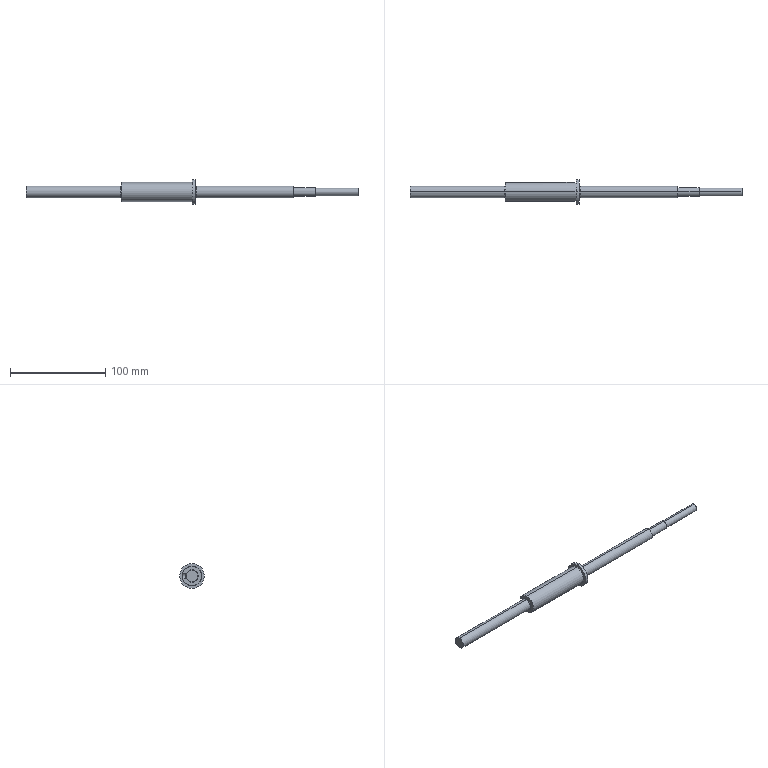Component | SolidWorks | LongAxis(Modified)-1 | 1 solid | 37 faces | box 349 x 26 x 26 mm | volume 50537 mm3 | cylinder 15 | plane 12 | torus 10 | commonest cylinder face diameters 12 x4 8 x2 26 x2 20 x2 9 x2 3 x2 6 x1 | material AISI 1045 Steel, Cold Drawn
STEP:
#1=CARTESIAN_POINT('',(-2.202,0.5951,13.465));
#2=VERTEX_POINT('',#1);
#3=CARTESIAN_POINT('',(-2.202,0.5951,14.016));
#4=VERTEX_POINT('',#3);
#5=CARTESIAN_POINT('',(-2.202,0.5951,13.74));
#6=DIRECTION('',(-1.,0.,0.));
#7=DIRECTION('',(0.,0.,1.));
#8=AXIS2_PLACEMENT_3D('',#5,#6,#7);
#9=CIRCLE('',#8,0.2756);
#10=EDGE_CURVE('',#2,#4,#9,.T.);
#11=ORIENTED_EDGE('',*,*,#10,.F.);
#12=CARTESIAN_POINT('',(-2.163,0.5951,13.504));
#13=VERTEX_POINT('',#12);
#14=CARTESIAN_POINT('',(-2.163,0.5951,13.465));
#15=DIRECTION('',(0.,1.,0.));
#16=DIRECTION('',(0.,0.,1.));
#17=AXIS2_PLACEMENT_3D('',#14,#15,#16);
#18=CIRCLE('',#17,0.03937);
#19=EDGE_CURVE('',#2,#13,#18,.T.);
#20=ORIENTED_EDGE('',*,*,#19,.T.);
#21=CARTESIAN_POINT('',(-2.163,0.5951,13.976));
#22=VERTEX_POINT('',#21);
#23=CARTESIAN_POINT('',(-2.163,0.5951,13.74));
#24=DIRECTION('',(1.,0.,0.));
#25=DIRECTION('',(0.,0.,1.));
#26=AXIS2_PLACEMENT_3D('',#23,#24,#25);
#27=CIRCLE('',#26,0.2362);
#28=EDGE_CURVE('',#22,#13,#27,.T.);
#29=ORIENTED_EDGE('',*,*,#28,.F.);
#30=CARTESIAN_POINT('',(-2.163,0.5951,14.016));
#31=DIRECTION('',(0.,-1.,0.));
#32=DIRECTION('',(0.,0.,-1.));
#33=AXIS2_PLACEMENT_3D('',#30,#31,#32);
#34=CIRCLE('',#33,0.03937);
#35=EDGE_CURVE('',#4,#22,#34,.T.);
#36=ORIENTED_EDGE('',*,*,#35,.F.);
#37=EDGE_LOOP('',(#11,#20,#29,#36));
#38=FACE_OUTER_BOUND('',#37,.T.);
#39=CARTESIAN_POINT('',(-2.163,0.5951,13.74));
#40=DIRECTION('',(-1.,0.,0.));
#41=DIRECTION('',(0.,0.,1.));
#42=AXIS2_PLACEMENT_3D('',#39,#40,#41);
#43=TOROIDAL_SURFACE('',#42,0.2756,0.03937);
#44=ADVANCED_FACE('',(#38),#43,.F.);
#45=CARTESIAN_POINT('',(1.853,0.5951,13.543));
#46=VERTEX_POINT('',#45);
#47=CARTESIAN_POINT('',(1.853,0.5951,13.937));
#48=VERTEX_POINT('',#47);
#49=CARTESIAN_POINT('',(1.853,0.5951,13.74));
#50=DIRECTION('',(-1.,0.,0.));
#51=DIRECTION('',(0.,0.,1.));
#52=AXIS2_PLACEMENT_3D('',#49,#50,#51);
#53=CIRCLE('',#52,0.1969);
#54=EDGE_CURVE('',#46,#48,#53,.T.);
#55=ORIENTED_EDGE('',*,*,#54,.F.);
#56=CARTESIAN_POINT('',(1.873,0.5951,13.563));
#57=VERTEX_POINT('',#56);
#58=CARTESIAN_POINT('',(1.873,0.5951,13.543));
#59=DIRECTION('',(0.,1.,0.));
#60=DIRECTION('',(0.,0.,1.));
#61=AXIS2_PLACEMENT_3D('',#58,#59,#60);
#62=CIRCLE('',#61,0.01969);
#63=EDGE_CURVE('',#46,#57,#62,.T.);
#64=ORIENTED_EDGE('',*,*,#63,.T.);
#65=CARTESIAN_POINT('',(1.873,0.5951,13.917));
#66=VERTEX_POINT('',#65);
#67=CARTESIAN_POINT('',(1.873,0.5951,13.74));
#68=DIRECTION('',(1.,0.,0.));
#69=DIRECTION('',(0.,0.,1.));
#70=AXIS2_PLACEMENT_3D('',#67,#68,#69);
#71=CIRCLE('',#70,0.1772);
#72=EDGE_CURVE('',#66,#57,#71,.T.);
#73=ORIENTED_EDGE('',*,*,#72,.F.);
#74=CARTESIAN_POINT('',(1.873,0.5951,13.937));
#75=DIRECTION('',(0.,-1.,0.));
#76=DIRECTION('',(0.,0.,-1.));
#77=AXIS2_PLACEMENT_3D('',#74,#75,#76);
#78=CIRCLE('',#77,0.01969);
#79=EDGE_CURVE('',#48,#66,#78,.T.);
#80=ORIENTED_EDGE('',*,*,#79,.F.);
#81=EDGE_LOOP('',(#55,#64,#73,#80));
#82=FACE_OUTER_BOUND('',#81,.T.);
#83=CARTESIAN_POINT('',(1.873,0.5951,13.74));
#84=DIRECTION('',(-1.,0.,0.));
#85=DIRECTION('',(0.,0.,1.));
#86=AXIS2_PLACEMENT_3D('',#83,#84,#85);
#87=TOROIDAL_SURFACE('',#86,0.1969,0.01969);
#88=ADVANCED_FACE('',(#82),#87,.F.);
#89=CARTESIAN_POINT('',(2.758,0.5951,13.563));
#90=VERTEX_POINT('',#89);
#91=CARTESIAN_POINT('',(2.758,0.5951,13.917));
#92=VERTEX_POINT('',#91);
#93=CARTESIAN_POINT('',(2.758,0.5951,13.74));
#94=DIRECTION('',(-1.,0.,0.));
#95=DIRECTION('',(0.,0.,1.));
#96=AXIS2_PLACEMENT_3D('',#93,#94,#95);
#97=CIRCLE('',#96,0.1772);
#98=EDGE_CURVE('',#90,#92,#97,.T.);
#99=ORIENTED_EDGE('',*,*,#98,.F.);
#100=CARTESIAN_POINT('',(2.778,0.5951,13.583));
#101=VERTEX_POINT('',#100);
#102=CARTESIAN_POINT('',(2.778,0.5951,13.563));
#103=DIRECTION('',(0.,1.,0.));
#104=DIRECTION('',(0.,0.,1.));
#105=AXIS2_PLACEMENT_3D('',#102,#103,#104);
#106=CIRCLE('',#105,0.01969);
#107=EDGE_CURVE('',#90,#101,#106,.T.);
#108=ORIENTED_EDGE('',*,*,#107,.T.);
#109=CARTESIAN_POINT('',(2.778,0.5951,13.898));
#110=VERTEX_POINT('',#109);
#111=CARTESIAN_POINT('',(2.778,0.5951,13.74));
#112=DIRECTION('',(1.,0.,0.));
#113=DIRECTION('',(0.,0.,1.));
#114=AXIS2_PLACEMENT_3D('',#111,#112,#113);
#115=CIRCLE('',#114,0.1575);
#116=EDGE_CURVE('',#110,#101,#115,.T.);
#117=ORIENTED_EDGE('',*,*,#116,.F.);
#118=CARTESIAN_POINT('',(2.778,0.5951,13.917));
#119=DIRECTION('',(0.,-1.,0.));
#120=DIRECTION('',(0.,0.,-1.));
#121=AXIS2_PLACEMENT_3D('',#118,#119,#120);
#122=CIRCLE('',#121,0.01969);
#123=EDGE_CURVE('',#92,#110,#122,.T.);
#124=ORIENTED_EDGE('',*,*,#123,.F.);
#125=EDGE_LOOP('',(#99,#108,#117,#124));
#126=FACE_OUTER_BOUND('',#125,.T.);
#127=CARTESIAN_POINT('',(2.778,0.5951,13.74));
#128=DIRECTION('',(-1.,0.,0.));
#129=DIRECTION('',(0.,0.,1.));
#130=AXIS2_PLACEMENT_3D('',#127,#128,#129);
#131=TOROIDAL_SURFACE('',#130,0.1772,0.01969);
#132=ADVANCED_FACE('',(#126),#131,.F.);
#133=CARTESIAN_POINT('',(-5.273,0.5951,13.996));
#134=VERTEX_POINT('',#133);
#135=CARTESIAN_POINT('',(-5.273,0.5951,13.484));
#136=VERTEX_POINT('',#135);
#137=CARTESIAN_POINT('',(-5.273,0.5951,13.74));
#138=DIRECTION('',(1.,0.,0.));
#139=DIRECTION('',(0.,0.,-1.));
#140=AXIS2_PLACEMENT_3D('',#137,#138,#139);
#141=CIRCLE('',#140,0.2559);
#142=EDGE_CURVE('',#134,#136,#141,.T.);
#143=ORIENTED_EDGE('',*,*,#142,.F.);
#144=CARTESIAN_POINT('',(-5.293,0.5951,13.976));
#145=VERTEX_POINT('',#144);
#146=CARTESIAN_POINT('',(-5.293,0.5951,13.996));
#147=DIRECTION('',(0.,1.,-0.));
#148=DIRECTION('',(0.,0.,1.));
#149=AXIS2_PLACEMENT_3D('',#146,#147,#148);
#150=CIRCLE('',#149,0.01969);
#151=EDGE_CURVE('',#134,#145,#150,.T.);
#152=ORIENTED_EDGE('',*,*,#151,.T.);
#153=CARTESIAN_POINT('',(-5.293,0.5951,13.504));
#154=VERTEX_POINT('',#153);
#155=CARTESIAN_POINT('',(-5.293,0.5951,13.74));
#156=DIRECTION('',(-1.,0.,0.));
#157=DIRECTION('',(0.,0.,-1.));
#158=AXIS2_PLACEMENT_3D('',#155,#156,#157);
#159=CIRCLE('',#158,0.2362);
#160=EDGE_CURVE('',#154,#145,#159,.T.);
#161=ORIENTED_EDGE('',*,*,#160,.F.);
#162=CARTESIAN_POINT('',(-5.293,0.5951,13.484));
#163=DIRECTION('',(0.,-1.,0.));
#164=DIRECTION('',(0.,0.,-1.));
#165=AXIS2_PLACEMENT_3D('',#162,#163,#164);
#166=CIRCLE('',#165,0.01969);
#167=EDGE_CURVE('',#136,#154,#166,.T.);
#168=ORIENTED_EDGE('',*,*,#167,.F.);
#169=EDGE_LOOP('',(#143,#152,#161,#168));
#170=FACE_OUTER_BOUND('',#169,.T.);
#171=CARTESIAN_POINT('',(-5.293,0.5951,13.74));
#172=DIRECTION('',(1.,0.,0.));
#173=DIRECTION('',(0.,0.,-1.));
#174=AXIS2_PLACEMENT_3D('',#171,#172,#173);
#175=TOROIDAL_SURFACE('',#174,0.2559,0.01969);
#176=ADVANCED_FACE('',(#170),#175,.F.);
#177=CARTESIAN_POINT('',(-2.32,0.5951,14.154));
#178=VERTEX_POINT('',#177);
#179=CARTESIAN_POINT('',(-2.32,0.5951,13.327));
#180=VERTEX_POINT('',#179);
#181=CARTESIAN_POINT('',(-2.32,0.5951,13.74));
#182=DIRECTION('',(1.,0.,0.));
#183=DIRECTION('',(0.,0.,-1.));
#184=AXIS2_PLACEMENT_3D('',#181,#182,#183);
#185=CIRCLE('',#184,0.4134);
#186=EDGE_CURVE('',#178,#180,#185,.T.);
#187=ORIENTED_EDGE('',*,*,#186,.F.);
#188=CARTESIAN_POINT('',(-2.34,0.5951,14.134));
#189=VERTEX_POINT('',#188);
#190=CARTESIAN_POINT('',(-2.34,0.5951,14.154));
#191=DIRECTION('',(0.,1.,-0.));
#192=DIRECTION('',(0.,0.,1.));
#193=AXIS2_PLACEMENT_3D('',#190,#191,#192);
#194=CIRCLE('',#193,0.01969);
#195=EDGE_CURVE('',#178,#189,#194,.T.);
#196=ORIENTED_EDGE('',*,*,#195,.T.);
#197=CARTESIAN_POINT('',(-2.34,0.5951,13.346));
#198=VERTEX_POINT('',#197);
#199=CARTESIAN_POINT('',(-2.34,0.5951,13.74));
#200=DIRECTION('',(-1.,0.,0.));
#201=DIRECTION('',(0.,0.,-1.));
#202=AXIS2_PLACEMENT_3D('',#199,#200,#201);
#203=CIRCLE('',#202,0.3937);
#204=EDGE_CURVE('',#198,#189,#203,.T.);
#205=ORIENTED_EDGE('',*,*,#204,.F.);
#206=CARTESIAN_POINT('',(-2.34,0.5951,13.327));
#207=DIRECTION('',(0.,-1.,0.));
#208=DIRECTION('',(0.,0.,-1.));
#209=AXIS2_PLACEMENT_3D('',#206,#207,#208);
#210=CIRCLE('',#209,0.01969);
#211=EDGE_CURVE('',#180,#198,#210,.T.);
#212=ORIENTED_EDGE('',*,*,#211,.F.);
#213=EDGE_LOOP('',(#187,#196,#205,#212));
#214=FACE_OUTER_BOUND('',#213,.T.);
#215=CARTESIAN_POINT('',(-2.34,0.5951,13.74));
#216=DIRECTION('',(1.,0.,0.));
#217=DIRECTION('',(0.,0.,-1.));
#218=AXIS2_PLACEMENT_3D('',#215,#216,#217);
#219=TOROIDAL_SURFACE('',#218,0.4134,0.01969);
#220=ADVANCED_FACE('',(#214),#219,.F.);
#221=CARTESIAN_POINT('',(4.53,0.5951,13.898));
#222=VERTEX_POINT('',#221);
#223=CARTESIAN_POINT('',(4.53,0.5951,13.583));
#224=VERTEX_POINT('',#223);
#225=CARTESIAN_POINT('',(4.53,0.5951,13.74));
#226=DIRECTION('',(-1.,0.,0.));
#227=DIRECTION('',(0.,0.,1.));
#228=AXIS2_PLACEMENT_3D('',#225,#226,#227);
#229=CIRCLE('',#228,0.1575);
#230=EDGE_CURVE('',#222,#224,#229,.T.);
#231=ORIENTED_EDGE('',*,*,#230,.T.);
#232=CARTESIAN_POINT('',(-9.21,0.5951,13.583));
#233=DIRECTION('',(-1.,0.,0.));
#234=VECTOR('',#233,39.37);
#235=LINE('',#232,#234);
#236=EDGE_CURVE('',#224,#101,#235,.T.);
#237=ORIENTED_EDGE('',*,*,#236,.T.);
#238=CARTESIAN_POINT('',(2.778,0.5951,13.74));
#239=DIRECTION('',(1.,0.,0.));
#240=DIRECTION('',(0.,0.,1.));
#241=AXIS2_PLACEMENT_3D('',#238,#239,#240);
#242=CIRCLE('',#241,0.1575);
#243=EDGE_CURVE('',#101,#110,#242,.T.);
#244=ORIENTED_EDGE('',*,*,#243,.T.);
#245=CARTESIAN_POINT('',(-9.21,0.5951,13.898));
#246=DIRECTION('',(-1.,0.,0.));
#247=VECTOR('',#246,39.37);
#248=LINE('',#245,#247);
#249=EDGE_CURVE('',#222,#110,#248,.T.);
#250=ORIENTED_EDGE('',*,*,#249,.F.);
#251=EDGE_LOOP('',(#231,#237,#244,#250));
#252=FACE_OUTER_BOUND('',#251,.T.);
#253=CARTESIAN_POINT('',(-9.21,0.5951,13.74));
#254=DIRECTION('',(-1.,0.,0.));
#255=DIRECTION('',(0.,0.,1.));
#256=AXIS2_PLACEMENT_3D('',#253,#254,#255);
#257=CYLINDRICAL_SURFACE('',#256,0.1575);
#258=ADVANCED_FACE('',(#252),#257,.T.);
#259=CARTESIAN_POINT('',(1.853,0.5951,13.976));
#260=VERTEX_POINT('',#259);
#261=CARTESIAN_POINT('',(1.853,0.5951,13.504));
#262=VERTEX_POINT('',#261);
#263=CARTESIAN_POINT('',(1.853,0.5951,13.74));
#264=DIRECTION('',(-1.,0.,0.));
#265=DIRECTION('',(0.,0.,1.));
#266=AXIS2_PLACEMENT_3D('',#263,#264,#265);
#267=CIRCLE('',#266,0.2362);
#268=EDGE_CURVE('',#260,#262,#267,.T.);
#269=ORIENTED_EDGE('',*,*,#268,.T.);
#270=CARTESIAN_POINT('',(-9.21,0.5951,13.504));
#271=DIRECTION('',(-1.,0.,0.));
#272=VECTOR('',#271,39.37);
#273=LINE('',#270,#272);
#274=EDGE_CURVE('',#262,#13,#273,.T.);
#275=ORIENTED_EDGE('',*,*,#274,.T.);
#276=CARTESIAN_POINT('',(-2.163,0.5951,13.74));
#277=DIRECTION('',(1.,0.,0.));
#278=DIRECTION('',(0.,0.,1.));
#279=AXIS2_PLACEMENT_3D('',#276,#277,#278);
#280=CIRCLE('',#279,0.2362);
#281=EDGE_CURVE('',#13,#22,#280,.T.);
#282=ORIENTED_EDGE('',*,*,#281,.T.);
#283=CARTESIAN_POINT('',(-9.21,0.5951,13.976));
#284=DIRECTION('',(-1.,0.,0.));
#285=VECTOR('',#284,39.37);
#286=LINE('',#283,#285);
#287=EDGE_CURVE('',#260,#22,#286,.T.);
#288=ORIENTED_EDGE('',*,*,#287,.F.);
#289=EDGE_LOOP('',(#269,#275,#282,#288));
#290=FACE_OUTER_BOUND('',#289,.T.);
#291=CARTESIAN_POINT('',(-9.21,0.5951,13.74));
#292=DIRECTION('',(-1.,0.,0.));
#293=DIRECTION('',(0.,0.,1.));
#294=AXIS2_PLACEMENT_3D('',#291,#292,#293);
#295=CYLINDRICAL_SURFACE('',#294,0.2362);
#296=ADVANCED_FACE('',(#290),#295,.T.);
#297=CARTESIAN_POINT('',(-2.202,0.5951,14.252));
#298=VERTEX_POINT('',#297);
#299=CARTESIAN_POINT('',(-2.202,0.5951,13.228));
#300=VERTEX_POINT('',#299);
#301=CARTESIAN_POINT('',(-2.202,0.5951,13.74));
#302=DIRECTION('',(-1.,0.,0.));
#303=DIRECTION('',(0.,0.,1.));
#304=AXIS2_PLACEMENT_3D('',#301,#302,#303);
#305=CIRCLE('',#304,0.5118);
#306=EDGE_CURVE('',#298,#300,#305,.T.);
#307=ORIENTED_EDGE('',*,*,#306,.T.);
#308=CARTESIAN_POINT('',(-2.32,0.5951,13.228));
#309=VERTEX_POINT('',#308);
#310=CARTESIAN_POINT('',(-9.21,0.5951,13.228));
#311=DIRECTION('',(-1.,0.,0.));
#312=VECTOR('',#311,39.37);
#313=LINE('',#310,#312);
#314=EDGE_CURVE('',#300,#309,#313,.T.);
#315=ORIENTED_EDGE('',*,*,#314,.T.);
#316=CARTESIAN_POINT('',(-2.32,0.5951,14.252));
#317=VERTEX_POINT('',#316);
#318=CARTESIAN_POINT('',(-2.32,0.5951,13.74));
#319=DIRECTION('',(-1.,0.,0.));
#320=DIRECTION('',(0.,0.,1.));
#321=AXIS2_PLACEMENT_3D('',#318,#319,#320);
#322=CIRCLE('',#321,0.5118);
#323=EDGE_CURVE('',#317,#309,#322,.T.);
#324=ORIENTED_EDGE('',*,*,#323,.F.);
#325=CARTESIAN_POINT('',(-9.21,0.5951,14.252));
#326=DIRECTION('',(-1.,0.,0.));
#327=VECTOR('',#326,39.37);
#328=LINE('',#325,#327);
#329=EDGE_CURVE('',#298,#317,#328,.T.);
#330=ORIENTED_EDGE('',*,*,#329,.F.);
#331=EDGE_LOOP('',(#307,#315,#324,#330));
#332=FACE_OUTER_BOUND('',#331,.T.);
#333=CARTESIAN_POINT('',(-9.21,0.5951,13.74));
#334=DIRECTION('',(-1.,0.,0.));
#335=DIRECTION('',(0.,0.,1.));
#336=AXIS2_PLACEMENT_3D('',#333,#334,#335);
#337=CYLINDRICAL_SURFACE('',#336,0.5118);
#338=ADVANCED_FACE('',(#332),#337,.T.);
#339=CARTESIAN_POINT('',(-5.293,0.5951,13.74));
#340=DIRECTION('',(-1.,0.,0.));
#341=DIRECTION('',(0.,0.,-1.));
#342=AXIS2_PLACEMENT_3D('',#339,#340,#341);
#343=CIRCLE('',#342,0.2362);
#344=EDGE_CURVE('',#145,#154,#343,.T.);
#345=ORIENTED_EDGE('',*,*,#344,.T.);
#346=CARTESIAN_POINT('',(-9.21,0.5951,13.504));
#347=VERTEX_POINT('',#346);
#348=CARTESIAN_POINT('',(-9.21,0.5951,13.504));
#349=DIRECTION('',(-1.,0.,0.));
#350=VECTOR('',#349,39.37);
#351=LINE('',#348,#350);
#352=EDGE_CURVE('',#154,#347,#351,.T.);
#353=ORIENTED_EDGE('',*,*,#352,.T.);
#354=CARTESIAN_POINT('',(-9.21,0.5951,13.976));
#355=VERTEX_POINT('',#354);
#356=CARTESIAN_POINT('',(-9.21,0.5951,13.74));
#357=DIRECTION('',(-1.,0.,0.));
#358=DIRECTION('',(0.,0.,1.));
#359=AXIS2_PLACEMENT_3D('',#356,#357,#358);
#360=CIRCLE('',#359,0.2362);
#361=EDGE_CURVE('',#355,#347,#360,.T.);
#362=ORIENTED_EDGE('',*,*,#361,.F.);
#363=CARTESIAN_POINT('',(-9.21,0.5951,13.976));
#364=DIRECTION('',(-1.,0.,0.));
#365=VECTOR('',#364,39.37);
#366=LINE('',#363,#365);
#367=EDGE_CURVE('',#145,#355,#366,.T.);
#368=ORIENTED_EDGE('',*,*,#367,.F.);
#369=EDGE_LOOP('',(#345,#353,#362,#368));
#370=FACE_OUTER_BOUND('',#369,.T.);
#371=CARTESIAN_POINT('',(-9.21,0.5951,13.74));
#372=DIRECTION('',(-1.,0.,0.));
#373=DIRECTION('',(0.,0.,1.));
#374=AXIS2_PLACEMENT_3D('',#371,#372,#373);
#375=CYLINDRICAL_SURFACE('',#374,0.2362);
#376=ADVANCED_FACE('',(#370),#375,.T.);
#377=CARTESIAN_POINT('',(-2.34,0.5951,13.74));
#378=DIRECTION('',(-1.,0.,0.));
#379=DIRECTION('',(0.,0.,-1.));
#380=AXIS2_PLACEMENT_3D('',#377,#378,#379);
#381=CIRCLE('',#380,0.3937);
#382=EDGE_CURVE('',#189,#198,#381,.T.);
#383=ORIENTED_EDGE('',*,*,#382,.T.);
#384=CARTESIAN_POINT('',(-5.273,0.5951,13.346));
#385=VERTEX_POINT('',#384);
#386=CARTESIAN_POINT('',(-9.21,0.5951,13.346));
#387=DIRECTION('',(-1.,0.,0.));
#388=VECTOR('',#387,39.37);
#389=LINE('',#386,#388);
#390=EDGE_CURVE('',#198,#385,#389,.T.);
#391=ORIENTED_EDGE('',*,*,#390,.T.);
#392=CARTESIAN_POINT('',(-5.273,0.9707,13.622));
#393=VERTEX_POINT('',#392);
#394=CARTESIAN_POINT('',(-5.273,0.5951,13.74));
#395=DIRECTION('',(-1.,0.,0.));
#396=DIRECTION('',(0.,0.,1.));
#397=AXIS2_PLACEMENT_3D('',#394,#395,#396);
#398=CIRCLE('',#397,0.3937);
#399=EDGE_CURVE('',#393,#385,#398,.T.);
#400=ORIENTED_EDGE('',*,*,#399,.F.);
#401=CARTESIAN_POINT('',(-2.911,0.9707,13.622));
#402=VERTEX_POINT('',#401);
#403=CARTESIAN_POINT('',(-9.21,0.9707,13.622));
#404=DIRECTION('',(-1.,0.,0.));
#405=VECTOR('',#404,39.37);
#406=LINE('',#403,#405);
#407=EDGE_CURVE('',#402,#393,#406,.T.);
#408=ORIENTED_EDGE('',*,*,#407,.F.);
#409=CARTESIAN_POINT('',(-2.911,0.9707,13.858));
#410=VERTEX_POINT('',#409);
#411=CARTESIAN_POINT('',(-2.911,0.9707,13.858));
#412=CARTESIAN_POINT('',(-2.903,0.9707,13.858));
#413=CARTESIAN_POINT('',(-2.895,0.9709,13.857));
#414=CARTESIAN_POINT('',(-2.88,0.9718,13.854));
#415=CARTESIAN_POINT('',(-2.873,0.9725,13.852));
#416=CARTESIAN_POINT('',(-2.858,0.9743,13.846));
#417=CARTESIAN_POINT('',(-2.852,0.9753,13.843));
#418=CARTESIAN_POINT('',(-2.839,0.9775,13.834));
#419=CARTESIAN_POINT('',(-2.833,0.9787,13.829));
#420=CARTESIAN_POINT('',(-2.817,0.9822,13.813));
#421=CARTESIAN_POINT('',(-2.808,0.9845,13.8));
#422=CARTESIAN_POINT('',(-2.799,0.987,13.778));
#423=CARTESIAN_POINT('',(-2.797,0.9877,13.771));
#424=CARTESIAN_POINT('',(-2.794,0.9886,13.756));
#425=CARTESIAN_POINT('',(-2.793,0.9888,13.748));
#426=CARTESIAN_POINT('',(-2.793,0.9888,13.733));
#427=CARTESIAN_POINT('',(-2.794,0.9886,13.725));
#428=CARTESIAN_POINT('',(-2.797,0.9877,13.709));
#429=CARTESIAN_POINT('',(-2.799,0.987,13.702));
#430=CARTESIAN_POINT('',(-2.805,0.9854,13.688));
#431=CARTESIAN_POINT('',(-2.808,0.9844,13.681));
#432=CARTESIAN_POINT('',(-2.817,0.9822,13.668));
#433=CARTESIAN_POINT('',(-2.822,0.981,13.662));
#434=CARTESIAN_POINT('',(-2.833,0.9787,13.651));
#435=CARTESIAN_POINT('',(-2.839,0.9775,13.646));
#436=CARTESIAN_POINT('',(-2.852,0.9753,13.638));
#437=CARTESIAN_POINT('',(-2.858,0.9743,13.634));
#438=CARTESIAN_POINT('',(-2.873,0.9726,13.628));
#439=CARTESIAN_POINT('',(-2.88,0.9719,13.626));
#440=CARTESIAN_POINT('',(-2.895,0.9709,13.623));
#441=CARTESIAN_POINT('',(-2.903,0.9707,13.622));
#442=CARTESIAN_POINT('',(-2.911,0.9707,13.622));
#443=B_SPLINE_CURVE_WITH_KNOTS('',3,(#411,#412,#413,#414,#415,#416,#417,#418,#419,#420,#421,#422,#423,#424,#425,#426,#427,#428,#429,#430,#431,#432,#433,#434,#435,#436,#437,#438,#439,#440,#441,#442),.UNSPECIFIED.,.F.,.F.,(4,2,2,2,2,2,2,2,2,2,2,2,2,2,2,4),(0.,0.0005894,0.001179,0.001768,0.002358,0.003536,0.004126,0.004715,0.005305,0.005894,0.006484,0.007073,0.007662,0.008252,0.008841,0.009431),.UNSPECIFIED.);
#444=EDGE_CURVE('',#410,#402,#443,.T.);
#445=ORIENTED_EDGE('',*,*,#444,.F.);
#446=CARTESIAN_POINT('',(-5.273,0.9707,13.858));
#447=VERTEX_POINT('',#446);
#448=CARTESIAN_POINT('',(-9.21,0.9707,13.858));
#449=DIRECTION('',(1.,0.,0.));
#450=VECTOR('',#449,39.37);
#451=LINE('',#448,#450);
#452=EDGE_CURVE('',#447,#410,#451,.T.);
#453=ORIENTED_EDGE('',*,*,#452,.F.);
#454=CARTESIAN_POINT('',(-5.273,0.5951,14.134));
#455=VERTEX_POINT('',#454);
#456=CARTESIAN_POINT('',(-5.273,0.5951,13.74));
#457=DIRECTION('',(-1.,0.,0.));
#458=DIRECTION('',(0.,0.,1.));
#459=AXIS2_PLACEMENT_3D('',#456,#457,#458);
#460=CIRCLE('',#459,0.3937);
#461=EDGE_CURVE('',#455,#447,#460,.T.);
#462=ORIENTED_EDGE('',*,*,#461,.F.);
#463=CARTESIAN_POINT('',(-9.21,0.5951,14.134));
#464=DIRECTION('',(-1.,0.,0.));
#465=VECTOR('',#464,39.37);
#466=LINE('',#463,#465);
#467=EDGE_CURVE('',#189,#455,#466,.T.);
#468=ORIENTED_EDGE('',*,*,#467,.F.);
#469=EDGE_LOOP('',(#383,#391,#400,#408,#445,#453,#462,#468));
#470=FACE_OUTER_BOUND('',#469,.T.);
#471=CARTESIAN_POINT('',(-9.21,0.5951,13.74));
#472=DIRECTION('',(-1.,0.,0.));
#473=DIRECTION('',(0.,0.,1.));
#474=AXIS2_PLACEMENT_3D('',#471,#472,#473);
#475=CYLINDRICAL_SURFACE('',#474,0.3937);
#476=ADVANCED_FACE('',(#470),#475,.T.);
#477=CARTESIAN_POINT('',(2.561,0.7621,13.799));
#478=VERTEX_POINT('',#477);
#479=CARTESIAN_POINT('',(2.561,0.7621,13.681));
#480=VERTEX_POINT('',#479);
#481=CARTESIAN_POINT('',(2.561,0.7621,13.799));
#482=CARTESIAN_POINT('',(2.565,0.7621,13.799));
#483=CARTESIAN_POINT('',(2.569,0.7623,13.799));
#484=CARTESIAN_POINT('',(2.577,0.7628,13.797));
#485=CARTESIAN_POINT('',(2.581,0.7632,13.796));
#486=CARTESIAN_POINT('',(2.591,0.7646,13.792));
#487=CARTESIAN_POINT('',(2.598,0.766,13.787));
#488=CARTESIAN_POINT('',(2.609,0.7686,13.777));
#489=CARTESIAN_POINT('',(2.613,0.7699,13.77));
#490=CARTESIAN_POINT('',(2.619,0.7717,13.756));
#491=CARTESIAN_POINT('',(2.621,0.7723,13.748));
#492=CARTESIAN_POINT('',(2.621,0.7723,13.736));
#493=CARTESIAN_POINT('',(2.62,0.7721,13.732));
#494=CARTESIAN_POINT('',(2.619,0.7716,13.725));
#495=CARTESIAN_POINT('',(2.618,0.7713,13.721));
#496=CARTESIAN_POINT('',(2.613,0.7699,13.71));
#497=CARTESIAN_POINT('',(2.609,0.7686,13.704));
#498=CARTESIAN_POINT('',(2.601,0.7666,13.696));
#499=CARTESIAN_POINT('',(2.598,0.766,13.693));
#500=CARTESIAN_POINT('',(2.591,0.7647,13.689));
#501=CARTESIAN_POINT('',(2.588,0.7642,13.687));
#502=CARTESIAN_POINT('',(2.577,0.7627,13.683));
#503=CARTESIAN_POINT('',(2.569,0.7621,13.681));
#504=CARTESIAN_POINT('',(2.561,0.7621,13.681));
#505=B_SPLINE_CURVE_WITH_KNOTS('',3,(#481,#482,#483,#484,#485,#486,#487,#488,#489,#490,#491,#492,#493,#494,#495,#496,#497,#498,#499,#500,#501,#502,#503,#504),.UNSPECIFIED.,.F.,.F.,(4,2,2,2,2,2,2,2,2,2,2,4),(0.,0.0002951,0.0005902,0.00118,0.001771,0.002361,0.002656,0.002951,0.003541,0.003836,0.004132,0.004722),.UNSPECIFIED.);
#506=EDGE_CURVE('',#478,#480,#505,.T.);
#507=ORIENTED_EDGE('',*,*,#506,.F.);
#508=CARTESIAN_POINT('',(2.05,0.7621,13.799));
#509=VERTEX_POINT('',#508);
#510=CARTESIAN_POINT('',(-9.21,0.7621,13.799));
#511=DIRECTION('',(1.,0.,0.));
#512=VECTOR('',#511,39.37);
#513=LINE('',#510,#512);
#514=EDGE_CURVE('',#509,#478,#513,.T.);
#515=ORIENTED_EDGE('',*,*,#514,.F.);
#516=CARTESIAN_POINT('',(2.05,0.7621,13.681));
#517=VERTEX_POINT('',#516);
#518=CARTESIAN_POINT('',(2.05,0.7621,13.681));
#519=CARTESIAN_POINT('',(2.046,0.7621,13.681));
#520=CARTESIAN_POINT('',(2.042,0.7623,13.681));
#521=CARTESIAN_POINT('',(2.034,0.7628,13.683));
#522=CARTESIAN_POINT('',(2.031,0.7632,13.684));
#523=CARTESIAN_POINT('',(2.02,0.7646,13.689));
#524=CARTESIAN_POINT('',(2.013,0.766,13.693));
#525=CARTESIAN_POINT('',(2.003,0.7686,13.704));
#526=CARTESIAN_POINT('',(1.998,0.7699,13.71));
#527=CARTESIAN_POINT('',(1.992,0.7717,13.725));
#528=CARTESIAN_POINT('',(1.991,0.7723,13.732));
#529=CARTESIAN_POINT('',(1.991,0.7723,13.744));
#530=CARTESIAN_POINT('',(1.991,0.7721,13.748));
#531=CARTESIAN_POINT('',(1.993,0.7716,13.756));
#532=CARTESIAN_POINT('',(1.994,0.7713,13.759));
#533=CARTESIAN_POINT('',(1.998,0.7699,13.77));
#534=CARTESIAN_POINT('',(2.002,0.7686,13.776));
#535=CARTESIAN_POINT('',(2.011,0.7666,13.785));
#536=CARTESIAN_POINT('',(2.014,0.766,13.787));
#537=CARTESIAN_POINT('',(2.02,0.7647,13.791));
#538=CARTESIAN_POINT('',(2.023,0.7642,13.793));
#539=CARTESIAN_POINT('',(2.034,0.7627,13.798));
#540=CARTESIAN_POINT('',(2.042,0.7621,13.799));
#541=CARTESIAN_POINT('',(2.05,0.7621,13.799));
#542=B_SPLINE_CURVE_WITH_KNOTS('',3,(#518,#519,#520,#521,#522,#523,#524,#525,#526,#527,#528,#529,#530,#531,#532,#533,#534,#535,#536,#537,#538,#539,#540,#541),.UNSPECIFIED.,.F.,.F.,(4,2,2,2,2,2,2,2,2,2,2,4),(0.,0.0002951,0.0005902,0.00118,0.001771,0.002361,0.002656,0.002951,0.003541,0.003836,0.004132,0.004722),.UNSPECIFIED.);
#543=EDGE_CURVE('',#517,#509,#542,.T.);
#544=ORIENTED_EDGE('',*,*,#543,.F.);
#545=CARTESIAN_POINT('',(-9.21,0.7621,13.681));
#546=DIRECTION('',(-1.,0.,0.));
#547=VECTOR('',#546,39.37);
#548=LINE('',#545,#547);
#549=EDGE_CURVE('',#480,#517,#548,.T.);
#550=ORIENTED_EDGE('',*,*,#549,.F.);
#551=EDGE_LOOP('',(#507,#515,#544,#550));
#552=FACE_BOUND('',#551,.T.);
#553=CARTESIAN_POINT('',(2.758,0.5951,13.74));
#554=DIRECTION('',(-1.,0.,0.));
#555=DIRECTION('',(0.,0.,1.));
#556=AXIS2_PLACEMENT_3D('',#553,#554,#555);
#557=CIRCLE('',#556,0.1772);
#558=EDGE_CURVE('',#92,#90,#557,.T.);
#559=ORIENTED_EDGE('',*,*,#558,.T.);
#560=CARTESIAN_POINT('',(-9.21,0.5951,13.563));
#561=DIRECTION('',(-1.,0.,0.));
#562=VECTOR('',#561,39.37);
#563=LINE('',#560,#562);
#564=EDGE_CURVE('',#90,#57,#563,.T.);
#565=ORIENTED_EDGE('',*,*,#564,.T.);
#566=CARTESIAN_POINT('',(1.873,0.5951,13.74));
#567=DIRECTION('',(1.,0.,0.));
#568=DIRECTION('',(0.,0.,1.));
#569=AXIS2_PLACEMENT_3D('',#566,#567,#568);
#570=CIRCLE('',#569,0.1772);
#571=EDGE_CURVE('',#57,#66,#570,.T.);
#572=ORIENTED_EDGE('',*,*,#571,.T.);
#573=CARTESIAN_POINT('',(-9.21,0.5951,13.917));
#574=DIRECTION('',(-1.,0.,0.));
#575=VECTOR('',#574,39.37);
#576=LINE('',#573,#575);
#577=EDGE_CURVE('',#92,#66,#576,.T.);
#578=ORIENTED_EDGE('',*,*,#577,.F.);
#579=EDGE_LOOP('',(#559,#565,#572,#578));
#580=FACE_OUTER_BOUND('',#579,.T.);
#581=CARTESIAN_POINT('',(-9.21,0.5951,13.74));
#582=DIRECTION('',(-1.,0.,0.));
#583=DIRECTION('',(0.,0.,1.));
#584=AXIS2_PLACEMENT_3D('',#581,#582,#583);
#585=CYLINDRICAL_SURFACE('',#584,0.1772);
#586=ADVANCED_FACE('',(#552,#580),#585,.T.);
#587=ORIENTED_EDGE('',*,*,#564,.F.);
#588=ORIENTED_EDGE('',*,*,#98,.T.);
#589=ORIENTED_EDGE('',*,*,#577,.T.);
#590=ORIENTED_EDGE('',*,*,#72,.T.);
#591=EDGE_LOOP('',(#587,#588,#589,#590));
#592=FACE_OUTER_BOUND('',#591,.T.);
#593=CARTESIAN_POINT('',(-9.21,0.5951,13.74));
#594=DIRECTION('',(-1.,0.,0.));
#595=DIRECTION('',(0.,0.,1.));
#596=AXIS2_PLACEMENT_3D('',#593,#594,#595);
#597=CYLINDRICAL_SURFACE('',#596,0.1772);
#598=ADVANCED_FACE('',(#592),#597,.T.);
#599=CARTESIAN_POINT('',(-5.273,0.851,13.622));
#600=VERTEX_POINT('',#599);
#601=CARTESIAN_POINT('',(-5.273,0.8313,13.622));
#602=DIRECTION('',(0.,-1.,0.));
#603=VECTOR('',#602,39.37);
#604=LINE('',#601,#603);
#605=EDGE_CURVE('',#393,#600,#604,.T.);
#606=ORIENTED_EDGE('',*,*,#605,.F.);
#607=ORIENTED_EDGE('',*,*,#399,.T.);
#608=CARTESIAN_POINT('',(-5.273,0.5951,13.74));
#609=DIRECTION('',(-1.,0.,0.));
#610=DIRECTION('',(0.,0.,1.));
#611=AXIS2_PLACEMENT_3D('',#608,#609,#610);
#612=CIRCLE('',#611,0.3937);
#613=EDGE_CURVE('',#385,#455,#612,.T.);
#614=ORIENTED_EDGE('',*,*,#613,.T.);
#615=ORIENTED_EDGE('',*,*,#461,.T.);
#616=CARTESIAN_POINT('',(-5.273,0.851,13.858));
#617=VERTEX_POINT('',#616);
#618=CARTESIAN_POINT('',(-5.273,0.8313,13.858));
#619=DIRECTION('',(0.,1.,0.));
#620=VECTOR('',#619,39.37);
#621=LINE('',#618,#620);
#622=EDGE_CURVE('',#617,#447,#621,.T.);
#623=ORIENTED_EDGE('',*,*,#622,.F.);
#624=CARTESIAN_POINT('',(-5.273,0.851,13.74));
#625=VERTEX_POINT('',#624);
#626=CARTESIAN_POINT('',(-5.273,0.851,13.74));
#627=DIRECTION('',(0.,0.,1.));
#628=VECTOR('',#627,39.37);
#629=LINE('',#626,#628);
#630=EDGE_CURVE('',#625,#617,#629,.T.);
#631=ORIENTED_EDGE('',*,*,#630,.F.);
#632=CARTESIAN_POINT('',(-5.273,0.5951,13.74));
#633=DIRECTION('',(1.,0.,0.));
#634=DIRECTION('',(0.,0.,-1.));
#635=AXIS2_PLACEMENT_3D('',#632,#633,#634);
#636=CIRCLE('',#635,0.2559);
#637=EDGE_CURVE('',#625,#134,#636,.T.);
#638=ORIENTED_EDGE('',*,*,#637,.T.);
#639=ORIENTED_EDGE('',*,*,#142,.T.);
#640=CARTESIAN_POINT('',(-5.273,0.5951,13.74));
#641=DIRECTION('',(1.,0.,0.));
#642=DIRECTION('',(0.,0.,-1.));
#643=AXIS2_PLACEMENT_3D('',#640,#641,#642);
#644=CIRCLE('',#643,0.2559);
#645=EDGE_CURVE('',#136,#625,#644,.T.);
#646=ORIENTED_EDGE('',*,*,#645,.T.);
#647=CARTESIAN_POINT('',(-5.273,0.851,13.74));
#648=DIRECTION('',(0.,0.,1.));
#649=VECTOR('',#648,39.37);
#650=LINE('',#647,#649);
#651=EDGE_CURVE('',#600,#625,#650,.T.);
#652=ORIENTED_EDGE('',*,*,#651,.F.);
#653=EDGE_LOOP('',(#606,#607,#614,#615,#623,#631,#638,#639,#646,#652));
#654=FACE_OUTER_BOUND('',#653,.T.);
#655=CARTESIAN_POINT('',(-5.273,0.8313,13.74));
#656=DIRECTION('',(1.,0.,0.));
#657=DIRECTION('',(0.,0.,-1.));
#658=AXIS2_PLACEMENT_3D('',#655,#656,#657);
#659=PLANE('',#658);
#660=ADVANCED_FACE('',(#654),#659,.F.);
#661=ORIENTED_EDGE('',*,*,#390,.F.);
#662=ORIENTED_EDGE('',*,*,#204,.T.);
#663=ORIENTED_EDGE('',*,*,#467,.T.);
#664=ORIENTED_EDGE('',*,*,#613,.F.);
#665=EDGE_LOOP('',(#661,#662,#663,#664));
#666=FACE_OUTER_BOUND('',#665,.T.);
#667=CARTESIAN_POINT('',(-9.21,0.5951,13.74));
#668=DIRECTION('',(-1.,0.,0.));
#669=DIRECTION('',(0.,0.,1.));
#670=AXIS2_PLACEMENT_3D('',#667,#668,#669);
#671=CYLINDRICAL_SURFACE('',#670,0.3937);
#672=ADVANCED_FACE('',(#666),#671,.T.);
#673=ORIENTED_EDGE('',*,*,#361,.T.);
#674=CARTESIAN_POINT('',(-9.21,0.5951,13.74));
#675=DIRECTION('',(-1.,0.,0.));
#676=DIRECTION('',(0.,0.,1.));
#677=AXIS2_PLACEMENT_3D('',#674,#675,#676);
#678=CIRCLE('',#677,0.2362);
#679=EDGE_CURVE('',#347,#355,#678,.T.);
#680=ORIENTED_EDGE('',*,*,#679,.T.);
#681=EDGE_LOOP('',(#673,#680));
#682=FACE_OUTER_BOUND('',#681,.T.);
#683=CARTESIAN_POINT('',(-9.21,0.5951,13.74));
#684=DIRECTION('',(1.,0.,0.));
#685=DIRECTION('',(0.,0.,-1.));
#686=AXIS2_PLACEMENT_3D('',#683,#684,#685);
#687=PLANE('',#686);
#688=ADVANCED_FACE('',(#682),#687,.F.);
#689=ORIENTED_EDGE('',*,*,#352,.F.);
#690=ORIENTED_EDGE('',*,*,#160,.T.);
#691=ORIENTED_EDGE('',*,*,#367,.T.);
#692=ORIENTED_EDGE('',*,*,#679,.F.);
#693=EDGE_LOOP('',(#689,#690,#691,#692));
#694=FACE_OUTER_BOUND('',#693,.T.);
#695=CARTESIAN_POINT('',(-9.21,0.5951,13.74));
#696=DIRECTION('',(-1.,0.,0.));
#697=DIRECTION('',(0.,0.,1.));
#698=AXIS2_PLACEMENT_3D('',#695,#696,#697);
#699=CYLINDRICAL_SURFACE('',#698,0.2362);
#700=ADVANCED_FACE('',(#694),#699,.T.);
#701=CARTESIAN_POINT('',(-2.32,0.5951,13.74));
#702=DIRECTION('',(1.,0.,0.));
#703=DIRECTION('',(0.,0.,-1.));
#704=AXIS2_PLACEMENT_3D('',#701,#702,#703);
#705=CIRCLE('',#704,0.4134);
#706=EDGE_CURVE('',#180,#178,#705,.T.);
#707=ORIENTED_EDGE('',*,*,#706,.T.);
#708=ORIENTED_EDGE('',*,*,#186,.T.);
#709=EDGE_LOOP('',(#707,#708));
#710=FACE_BOUND('',#709,.T.);
#711=ORIENTED_EDGE('',*,*,#323,.T.);
#712=CARTESIAN_POINT('',(-2.32,0.5951,13.74));
#713=DIRECTION('',(-1.,0.,0.));
#714=DIRECTION('',(0.,0.,1.));
#715=AXIS2_PLACEMENT_3D('',#712,#713,#714);
#716=CIRCLE('',#715,0.5118);
#717=EDGE_CURVE('',#309,#317,#716,.T.);
#718=ORIENTED_EDGE('',*,*,#717,.T.);
#719=EDGE_LOOP('',(#711,#718));
#720=FACE_OUTER_BOUND('',#719,.T.);
#721=CARTESIAN_POINT('',(-2.32,0.9888,13.74));
#722=DIRECTION('',(1.,0.,0.));
#723=DIRECTION('',(0.,0.,-1.));
#724=AXIS2_PLACEMENT_3D('',#721,#722,#723);
#725=PLANE('',#724);
#726=ADVANCED_FACE('',(#710,#720),#725,.F.);
#727=ORIENTED_EDGE('',*,*,#314,.F.);
#728=CARTESIAN_POINT('',(-2.202,0.5951,13.74));
#729=DIRECTION('',(-1.,0.,0.));
#730=DIRECTION('',(0.,0.,1.));
#731=AXIS2_PLACEMENT_3D('',#728,#729,#730);
#732=CIRCLE('',#731,0.5118);
#733=EDGE_CURVE('',#300,#298,#732,.T.);
#734=ORIENTED_EDGE('',*,*,#733,.T.);
#735=ORIENTED_EDGE('',*,*,#329,.T.);
#736=ORIENTED_EDGE('',*,*,#717,.F.);
#737=EDGE_LOOP('',(#727,#734,#735,#736));
#738=FACE_OUTER_BOUND('',#737,.T.);
#739=CARTESIAN_POINT('',(-9.21,0.5951,13.74));
#740=DIRECTION('',(-1.,0.,0.));
#741=DIRECTION('',(0.,0.,1.));
#742=AXIS2_PLACEMENT_3D('',#739,#740,#741);
#743=CYLINDRICAL_SURFACE('',#742,0.5118);
#744=ADVANCED_FACE('',(#738),#743,.T.);
#745=CARTESIAN_POINT('',(-2.202,0.5951,13.74));
#746=DIRECTION('',(-1.,0.,0.));
#747=DIRECTION('',(0.,0.,1.));
#748=AXIS2_PLACEMENT_3D('',#745,#746,#747);
#749=CIRCLE('',#748,0.2756);
#750=EDGE_CURVE('',#4,#2,#749,.T.);
#751=ORIENTED_EDGE('',*,*,#750,.T.);
#752=ORIENTED_EDGE('',*,*,#10,.T.);
#753=EDGE_LOOP('',(#751,#752));
#754=FACE_BOUND('',#753,.T.);
#755=ORIENTED_EDGE('',*,*,#306,.F.);
#756=ORIENTED_EDGE('',*,*,#733,.F.);
#757=EDGE_LOOP('',(#755,#756));
#758=FACE_OUTER_BOUND('',#757,.T.);
#759=CARTESIAN_POINT('',(-2.202,1.107,13.74));
#760=DIRECTION('',(-1.,0.,0.));
#761=DIRECTION('',(0.,0.,1.));
#762=AXIS2_PLACEMENT_3D('',#759,#760,#761);
#763=PLANE('',#762);
#764=ADVANCED_FACE('',(#754,#758),#763,.F.);
#765=ORIENTED_EDGE('',*,*,#274,.F.);
#766=CARTESIAN_POINT('',(1.853,0.5951,13.74));
#767=DIRECTION('',(-1.,0.,0.));
#768=DIRECTION('',(0.,0.,1.));
#769=AXIS2_PLACEMENT_3D('',#766,#767,#768);
#770=CIRCLE('',#769,0.2362);
#771=EDGE_CURVE('',#262,#260,#770,.T.);
#772=ORIENTED_EDGE('',*,*,#771,.T.);
#773=ORIENTED_EDGE('',*,*,#287,.T.);
#774=ORIENTED_EDGE('',*,*,#28,.T.);
#775=EDGE_LOOP('',(#765,#772,#773,#774));
#776=FACE_OUTER_BOUND('',#775,.T.);
#777=CARTESIAN_POINT('',(-9.21,0.5951,13.74));
#778=DIRECTION('',(-1.,0.,0.));
#779=DIRECTION('',(0.,0.,1.));
#780=AXIS2_PLACEMENT_3D('',#777,#778,#779);
#781=CYLINDRICAL_SURFACE('',#780,0.2362);
#782=ADVANCED_FACE('',(#776),#781,.T.);
#783=CARTESIAN_POINT('',(1.853,0.5951,13.74));
#784=DIRECTION('',(-1.,0.,0.));
#785=DIRECTION('',(0.,0.,1.));
#786=AXIS2_PLACEMENT_3D('',#783,#784,#785);
#787=CIRCLE('',#786,0.1969);
#788=EDGE_CURVE('',#48,#46,#787,.T.);
#789=ORIENTED_EDGE('',*,*,#788,.T.);
#790=ORIENTED_EDGE('',*,*,#54,.T.);
#791=EDGE_LOOP('',(#789,#790));
#792=FACE_BOUND('',#791,.T.);
#793=ORIENTED_EDGE('',*,*,#268,.F.);
#794=ORIENTED_EDGE('',*,*,#771,.F.);
#795=EDGE_LOOP('',(#793,#794));
#796=FACE_OUTER_BOUND('',#795,.T.);
#797=CARTESIAN_POINT('',(1.853,0.8313,13.74));
#798=DIRECTION('',(-1.,0.,0.));
#799=DIRECTION('',(0.,0.,1.));
#800=AXIS2_PLACEMENT_3D('',#797,#798,#799);
#801=PLANE('',#800);
#802=ADVANCED_FACE('',(#792,#796),#801,.F.);
#803=ORIENTED_EDGE('',*,*,#236,.F.);
#804=CARTESIAN_POINT('',(4.53,0.5951,13.74));
#805=DIRECTION('',(-1.,0.,0.));
#806=DIRECTION('',(0.,0.,1.));
#807=AXIS2_PLACEMENT_3D('',#804,#805,#806);
#808=CIRCLE('',#807,0.1575);
#809=EDGE_CURVE('',#224,#222,#808,.T.);
#810=ORIENTED_EDGE('',*,*,#809,.T.);
#811=ORIENTED_EDGE('',*,*,#249,.T.);
#812=ORIENTED_EDGE('',*,*,#116,.T.);
#813=EDGE_LOOP('',(#803,#810,#811,#812));
#814=FACE_OUTER_BOUND('',#813,.T.);
#815=CARTESIAN_POINT('',(-9.21,0.5951,13.74));
#816=DIRECTION('',(-1.,0.,0.));
#817=DIRECTION('',(0.,0.,1.));
#818=AXIS2_PLACEMENT_3D('',#815,#816,#817);
#819=CYLINDRICAL_SURFACE('',#818,0.1575);
#820=ADVANCED_FACE('',(#814),#819,.T.);
#821=ORIENTED_EDGE('',*,*,#230,.F.);
#822=ORIENTED_EDGE('',*,*,#809,.F.);
#823=EDGE_LOOP('',(#821,#822));
#824=FACE_OUTER_BOUND('',#823,.T.);
#825=CARTESIAN_POINT('',(4.53,0.7526,13.74));
#826=DIRECTION('',(-1.,0.,0.));
#827=DIRECTION('',(0.,0.,1.));
#828=AXIS2_PLACEMENT_3D('',#825,#826,#827);
#829=PLANE('',#828);
#830=ADVANCED_FACE('',(#824),#829,.F.);
#831=ORIENTED_EDGE('',*,*,#195,.F.);
#832=ORIENTED_EDGE('',*,*,#706,.F.);
#833=ORIENTED_EDGE('',*,*,#211,.T.);
#834=ORIENTED_EDGE('',*,*,#382,.F.);
#835=EDGE_LOOP('',(#831,#832,#833,#834));
#836=FACE_OUTER_BOUND('',#835,.T.);
#837=CARTESIAN_POINT('',(-2.34,0.5951,13.74));
#838=DIRECTION('',(1.,0.,0.));
#839=DIRECTION('',(0.,0.,-1.));
#840=AXIS2_PLACEMENT_3D('',#837,#838,#839);
#841=TOROIDAL_SURFACE('',#840,0.4134,0.01969);
#842=ADVANCED_FACE('',(#836),#841,.F.);
#843=ORIENTED_EDGE('',*,*,#151,.F.);
#844=ORIENTED_EDGE('',*,*,#637,.F.);
#845=ORIENTED_EDGE('',*,*,#645,.F.);
#846=ORIENTED_EDGE('',*,*,#167,.T.);
#847=ORIENTED_EDGE('',*,*,#344,.F.);
#848=EDGE_LOOP('',(#843,#844,#845,#846,#847));
#849=FACE_OUTER_BOUND('',#848,.T.);
#850=CARTESIAN_POINT('',(-5.293,0.5951,13.74));
#851=DIRECTION('',(1.,0.,0.));
#852=DIRECTION('',(0.,0.,-1.));
#853=AXIS2_PLACEMENT_3D('',#850,#851,#852);
#854=TOROIDAL_SURFACE('',#853,0.2559,0.01969);
#855=ADVANCED_FACE('',(#849),#854,.F.);
#856=ORIENTED_EDGE('',*,*,#107,.F.);
#857=ORIENTED_EDGE('',*,*,#558,.F.);
#858=ORIENTED_EDGE('',*,*,#123,.T.);
#859=ORIENTED_EDGE('',*,*,#243,.F.);
#860=EDGE_LOOP('',(#856,#857,#858,#859));
#861=FACE_OUTER_BOUND('',#860,.T.);
#862=CARTESIAN_POINT('',(2.778,0.5951,13.74));
#863=DIRECTION('',(-1.,0.,0.));
#864=DIRECTION('',(0.,0.,1.));
#865=AXIS2_PLACEMENT_3D('',#862,#863,#864);
#866=TOROIDAL_SURFACE('',#865,0.1772,0.01969);
#867=ADVANCED_FACE('',(#861),#866,.F.);
#868=ORIENTED_EDGE('',*,*,#63,.F.);
#869=ORIENTED_EDGE('',*,*,#788,.F.);
#870=ORIENTED_EDGE('',*,*,#79,.T.);
#871=ORIENTED_EDGE('',*,*,#571,.F.);
#872=EDGE_LOOP('',(#868,#869,#870,#871));
#873=FACE_OUTER_BOUND('',#872,.T.);
#874=CARTESIAN_POINT('',(1.873,0.5951,13.74));
#875=DIRECTION('',(-1.,0.,0.));
#876=DIRECTION('',(0.,0.,1.));
#877=AXIS2_PLACEMENT_3D('',#874,#875,#876);
#878=TOROIDAL_SURFACE('',#877,0.1969,0.01969);
#879=ADVANCED_FACE('',(#873),#878,.F.);
#880=ORIENTED_EDGE('',*,*,#19,.F.);
#881=ORIENTED_EDGE('',*,*,#750,.F.);
#882=ORIENTED_EDGE('',*,*,#35,.T.);
#883=ORIENTED_EDGE('',*,*,#281,.F.);
#884=EDGE_LOOP('',(#880,#881,#882,#883));
#885=FACE_OUTER_BOUND('',#884,.T.);
#886=CARTESIAN_POINT('',(-2.163,0.5951,13.74));
#887=DIRECTION('',(-1.,0.,0.));
#888=DIRECTION('',(0.,0.,1.));
#889=AXIS2_PLACEMENT_3D('',#886,#887,#888);
#890=TOROIDAL_SURFACE('',#889,0.2756,0.03937);
#891=ADVANCED_FACE('',(#885),#890,.F.);
#892=ORIENTED_EDGE('',*,*,#444,.T.);
#893=CARTESIAN_POINT('',(-2.911,0.851,13.622));
#894=VERTEX_POINT('',#893);
#895=CARTESIAN_POINT('',(-2.911,1.245,13.622));
#896=DIRECTION('',(0.,-1.,0.));
#897=VECTOR('',#896,39.37);
#898=LINE('',#895,#897);
#899=EDGE_CURVE('',#402,#894,#898,.T.);
#900=ORIENTED_EDGE('',*,*,#899,.T.);
#901=CARTESIAN_POINT('',(-2.911,0.851,13.858));
#902=VERTEX_POINT('',#901);
#903=CARTESIAN_POINT('',(-2.911,0.851,13.74));
#904=DIRECTION('',(0.,1.,0.));
#905=DIRECTION('',(0.,0.,1.));
#906=AXIS2_PLACEMENT_3D('',#903,#904,#905);
#907=CIRCLE('',#906,0.1181);
#908=EDGE_CURVE('',#902,#894,#907,.T.);
#909=ORIENTED_EDGE('',*,*,#908,.F.);
#910=CARTESIAN_POINT('',(-2.911,1.245,13.858));
#911=DIRECTION('',(0.,-1.,0.));
#912=VECTOR('',#911,39.37);
#913=LINE('',#910,#912);
#914=EDGE_CURVE('',#410,#902,#913,.T.);
#915=ORIENTED_EDGE('',*,*,#914,.F.);
#916=EDGE_LOOP('',(#892,#900,#909,#915));
#917=FACE_OUTER_BOUND('',#916,.T.);
#918=CARTESIAN_POINT('',(-2.911,1.245,13.74));
#919=DIRECTION('',(0.,-1.,0.));
#920=DIRECTION('',(0.,0.,-1.));
#921=AXIS2_PLACEMENT_3D('',#918,#919,#920);
#922=CYLINDRICAL_SURFACE('',#921,0.1181);
#923=ADVANCED_FACE('',(#917),#922,.F.);
#924=ORIENTED_EDGE('',*,*,#605,.T.);
#925=CARTESIAN_POINT('',(-5.69,0.851,13.622));
#926=DIRECTION('',(-1.,0.,0.));
#927=VECTOR('',#926,39.37);
#928=LINE('',#925,#927);
#929=EDGE_CURVE('',#894,#600,#928,.T.);
#930=ORIENTED_EDGE('',*,*,#929,.F.);
#931=ORIENTED_EDGE('',*,*,#899,.F.);
#932=ORIENTED_EDGE('',*,*,#407,.T.);
#933=EDGE_LOOP('',(#924,#930,#931,#932));
#934=FACE_OUTER_BOUND('',#933,.T.);
#935=CARTESIAN_POINT('',(-5.69,1.245,13.622));
#936=DIRECTION('',(0.,0.,1.));
#937=DIRECTION('',(1.,0.,0.));
#938=AXIS2_PLACEMENT_3D('',#935,#936,#937);
#939=PLANE('',#938);
#940=ADVANCED_FACE('',(#934),#939,.T.);
#941=ORIENTED_EDGE('',*,*,#622,.T.);
#942=ORIENTED_EDGE('',*,*,#452,.T.);
#943=ORIENTED_EDGE('',*,*,#914,.T.);
#944=CARTESIAN_POINT('',(-5.69,0.851,13.858));
#945=DIRECTION('',(1.,0.,0.));
#946=VECTOR('',#945,39.37);
#947=LINE('',#944,#946);
#948=EDGE_CURVE('',#617,#902,#947,.T.);
#949=ORIENTED_EDGE('',*,*,#948,.F.);
#950=EDGE_LOOP('',(#941,#942,#943,#949));
#951=FACE_OUTER_BOUND('',#950,.T.);
#952=CARTESIAN_POINT('',(-5.69,1.245,13.858));
#953=DIRECTION('',(0.,0.,-1.));
#954=DIRECTION('',(-1.,0.,0.));
#955=AXIS2_PLACEMENT_3D('',#952,#953,#954);
#956=PLANE('',#955);
#957=ADVANCED_FACE('',(#951),#956,.T.);
#958=ORIENTED_EDGE('',*,*,#651,.T.);
#959=ORIENTED_EDGE('',*,*,#630,.T.);
#960=ORIENTED_EDGE('',*,*,#948,.T.);
#961=ORIENTED_EDGE('',*,*,#908,.T.);
#962=ORIENTED_EDGE('',*,*,#929,.T.);
#963=EDGE_LOOP('',(#958,#959,#960,#961,#962));
#964=FACE_OUTER_BOUND('',#963,.T.);
#965=CARTESIAN_POINT('',(-2.911,0.851,13.74));
#966=DIRECTION('',(0.,1.,0.));
#967=DIRECTION('',(0.,0.,1.));
#968=AXIS2_PLACEMENT_3D('',#965,#966,#967);
#969=PLANE('',#968);
#970=ADVANCED_FACE('',(#964),#969,.T.);
#971=ORIENTED_EDGE('',*,*,#506,.T.);
#972=CARTESIAN_POINT('',(2.561,0.7132,13.681));
#973=VERTEX_POINT('',#972);
#974=CARTESIAN_POINT('',(2.561,1.107,13.681));
#975=DIRECTION('',(0.,-1.,0.));
#976=VECTOR('',#975,39.37);
#977=LINE('',#974,#976);
#978=EDGE_CURVE('',#480,#973,#977,.T.);
#979=ORIENTED_EDGE('',*,*,#978,.T.);
#980=CARTESIAN_POINT('',(2.561,0.7132,13.799));
#981=VERTEX_POINT('',#980);
#982=CARTESIAN_POINT('',(2.561,0.7132,13.74));
#983=DIRECTION('',(0.,1.,0.));
#984=DIRECTION('',(0.,0.,1.));
#985=AXIS2_PLACEMENT_3D('',#982,#983,#984);
#986=CIRCLE('',#985,0.05906);
#987=EDGE_CURVE('',#981,#973,#986,.T.);
#988=ORIENTED_EDGE('',*,*,#987,.F.);
#989=CARTESIAN_POINT('',(2.561,1.107,13.799));
#990=DIRECTION('',(0.,-1.,0.));
#991=VECTOR('',#990,39.37);
#992=LINE('',#989,#991);
#993=EDGE_CURVE('',#478,#981,#992,.T.);
#994=ORIENTED_EDGE('',*,*,#993,.F.);
#995=EDGE_LOOP('',(#971,#979,#988,#994));
#996=FACE_OUTER_BOUND('',#995,.T.);
#997=CARTESIAN_POINT('',(2.561,1.107,13.74));
#998=DIRECTION('',(0.,-1.,0.));
#999=DIRECTION('',(0.,0.,-1.));
#1000=AXIS2_PLACEMENT_3D('',#997,#998,#999);
#1001=CYLINDRICAL_SURFACE('',#1000,0.05906);
#1002=ADVANCED_FACE('',(#996),#1001,.F.);
#1003=ORIENTED_EDGE('',*,*,#549,.T.);
#1004=CARTESIAN_POINT('',(2.05,0.7132,13.681));
#1005=VERTEX_POINT('',#1004);
#1006=CARTESIAN_POINT('',(2.05,1.107,13.681));
#1007=DIRECTION('',(0.,-1.,0.));
#1008=VECTOR('',#1007,39.37);
#1009=LINE('',#1006,#1008);
#1010=EDGE_CURVE('',#517,#1005,#1009,.T.);
#1011=ORIENTED_EDGE('',*,*,#1010,.T.);
#1012=CARTESIAN_POINT('',(2.05,0.7132,13.681));
#1013=DIRECTION('',(-1.,0.,0.));
#1014=VECTOR('',#1013,39.37);
#1015=LINE('',#1012,#1014);
#1016=EDGE_CURVE('',#973,#1005,#1015,.T.);
#1017=ORIENTED_EDGE('',*,*,#1016,.F.);
#1018=ORIENTED_EDGE('',*,*,#978,.F.);
#1019=EDGE_LOOP('',(#1003,#1011,#1017,#1018));
#1020=FACE_OUTER_BOUND('',#1019,.T.);
#1021=CARTESIAN_POINT('',(2.05,1.107,13.681));
#1022=DIRECTION('',(0.,0.,1.));
#1023=DIRECTION('',(1.,0.,0.));
#1024=AXIS2_PLACEMENT_3D('',#1021,#1022,#1023);
#1025=PLANE('',#1024);
#1026=ADVANCED_FACE('',(#1020),#1025,.T.);
#1027=ORIENTED_EDGE('',*,*,#543,.T.);
#1028=CARTESIAN_POINT('',(2.05,0.7132,13.799));
#1029=VERTEX_POINT('',#1028);
#1030=CARTESIAN_POINT('',(2.05,1.107,13.799));
#1031=DIRECTION('',(0.,-1.,0.));
#1032=VECTOR('',#1031,39.37);
#1033=LINE('',#1030,#1032);
#1034=EDGE_CURVE('',#509,#1029,#1033,.T.);
#1035=ORIENTED_EDGE('',*,*,#1034,.T.);
#1036=CARTESIAN_POINT('',(2.05,0.7132,13.74));
#1037=DIRECTION('',(0.,1.,0.));
#1038=DIRECTION('',(0.,0.,1.));
#1039=AXIS2_PLACEMENT_3D('',#1036,#1037,#1038);
#1040=CIRCLE('',#1039,0.05906);
#1041=EDGE_CURVE('',#1005,#1029,#1040,.T.);
#1042=ORIENTED_EDGE('',*,*,#1041,.F.);
#1043=ORIENTED_EDGE('',*,*,#1010,.F.);
#1044=EDGE_LOOP('',(#1027,#1035,#1042,#1043));
#1045=FACE_OUTER_BOUND('',#1044,.T.);
#1046=CARTESIAN_POINT('',(2.05,1.107,13.74));
#1047=DIRECTION('',(0.,-1.,0.));
#1048=DIRECTION('',(0.,0.,-1.));
#1049=AXIS2_PLACEMENT_3D('',#1046,#1047,#1048);
#1050=CYLINDRICAL_SURFACE('',#1049,0.05906);
#1051=ADVANCED_FACE('',(#1045),#1050,.F.);
#1052=ORIENTED_EDGE('',*,*,#514,.T.);
#1053=ORIENTED_EDGE('',*,*,#993,.T.);
#1054=CARTESIAN_POINT('',(2.05,0.7132,13.799));
#1055=DIRECTION('',(1.,0.,0.));
#1056=VECTOR('',#1055,39.37);
#1057=LINE('',#1054,#1056);
#1058=EDGE_CURVE('',#1029,#981,#1057,.T.);
#1059=ORIENTED_EDGE('',*,*,#1058,.F.);
#1060=ORIENTED_EDGE('',*,*,#1034,.F.);
#1061=EDGE_LOOP('',(#1052,#1053,#1059,#1060));
#1062=FACE_OUTER_BOUND('',#1061,.T.);
#1063=CARTESIAN_POINT('',(2.05,1.107,13.799));
#1064=DIRECTION('',(0.,0.,-1.));
#1065=DIRECTION('',(-1.,0.,0.));
#1066=AXIS2_PLACEMENT_3D('',#1063,#1064,#1065);
#1067=PLANE('',#1066);
#1068=ADVANCED_FACE('',(#1062),#1067,.T.);
#1069=ORIENTED_EDGE('',*,*,#987,.T.);
#1070=ORIENTED_EDGE('',*,*,#1016,.T.);
#1071=ORIENTED_EDGE('',*,*,#1041,.T.);
#1072=ORIENTED_EDGE('',*,*,#1058,.T.);
#1073=EDGE_LOOP('',(#1069,#1070,#1071,#1072));
#1074=FACE_OUTER_BOUND('',#1073,.T.);
#1075=CARTESIAN_POINT('',(2.561,0.7132,13.74));
#1076=DIRECTION('',(0.,1.,0.));
#1077=DIRECTION('',(0.,0.,1.));
#1078=AXIS2_PLACEMENT_3D('',#1075,#1076,#1077);
#1079=PLANE('',#1078);
#1080=ADVANCED_FACE('',(#1074),#1079,.T.);
#1081=CLOSED_SHELL('',(#44,#88,#132,#176,#220,#258,#296,#338,#376,#476,#586,#598,#660,#672,#688,#700,#726,#744,#764,#782,#802,#820,#830,#842,#855,#867,#879,#891,#923,#940,#957,#970,#1002,#1026,#1051,#1068,#1080));
#1082=MANIFOLD_SOLID_BREP('',#1081);
#1083=CARTESIAN_POINT('',(0.,0.,0.));
#1084=DIRECTION('',(0.,0.,1.));
#1085=DIRECTION('',(1.,0.,0.));
#1086=AXIS2_PLACEMENT_3D('',#1083,#1084,#1085);
#1087=(LENGTH_UNIT()NAMED_UNIT(*)SI_UNIT($,.METRE.));
#1088=LENGTH_MEASURE_WITH_UNIT(LENGTH_MEASURE(0.0254),#1087);
#1089=DIMENSIONAL_EXPONENTS(1.,0.,0.,0.,0.,0.,0.);
#1090=(CONVERSION_BASED_UNIT('',#1088)LENGTH_UNIT()NAMED_UNIT(#1089));
#1091=UNCERTAINTY_MEASURE_WITH_UNIT(LENGTH_MEASURE(0.00001),#1090,'','');
#1092=(NAMED_UNIT(*)PLANE_ANGLE_UNIT()SI_UNIT($,.RADIAN.));
#1093=(NAMED_UNIT(*)SI_UNIT($,.STERADIAN.)SOLID_ANGLE_UNIT());
#1094=(GEOMETRIC_REPRESENTATION_CONTEXT(3)GLOBAL_UNCERTAINTY_ASSIGNED_CONTEXT((#1091))GLOBAL_UNIT_ASSIGNED_CONTEXT((#1090,#1092,#1093))REPRESENTATION_CONTEXT('',''));
#1095=ADVANCED_BREP_SHAPE_REPRESENTATION('',(#1082,#1086),#1094);
#1096=COLOUR_RGB('',0.7922,0.8196,0.9333);
#1097=FILL_AREA_STYLE_COLOUR('',#1096);
#1098=FILL_AREA_STYLE('',(#1097));
#1099=SURFACE_STYLE_FILL_AREA(#1098);
#1100=SURFACE_SIDE_STYLE('',(#1099));
#1101=SURFACE_STYLE_USAGE(.BOTH.,#1100);
#1102=PRESENTATION_STYLE_ASSIGNMENT((#1101));
#1103=STYLED_ITEM('',(#1102),#1082);
#1104=(LENGTH_UNIT()NAMED_UNIT(*)SI_UNIT($,.METRE.));
#1105=LENGTH_MEASURE_WITH_UNIT(LENGTH_MEASURE(0.0254),#1104);
#1106=DIMENSIONAL_EXPONENTS(1.,0.,0.,0.,0.,0.,0.);
#1107=(CONVERSION_BASED_UNIT('',#1105)LENGTH_UNIT()NAMED_UNIT(#1106));
#1108=UNCERTAINTY_MEASURE_WITH_UNIT(LENGTH_MEASURE(0.00001),#1107,'','');
#1109=(NAMED_UNIT(*)PLANE_ANGLE_UNIT()SI_UNIT($,.RADIAN.));
#1110=(NAMED_UNIT(*)SI_UNIT($,.STERADIAN.)SOLID_ANGLE_UNIT());
#1111=(GEOMETRIC_REPRESENTATION_CONTEXT(3)GLOBAL_UNCERTAINTY_ASSIGNED_CONTEXT((#1108))GLOBAL_UNIT_ASSIGNED_CONTEXT((#1107,#1109,#1110))REPRESENTATION_CONTEXT('',''));
#1112=MECHANICAL_DESIGN_GEOMETRIC_PRESENTATION_REPRESENTATION('',(#1103),#1111);
#1113=PRESENTATION_LAYER_ASSIGNMENT('','',(#1103));